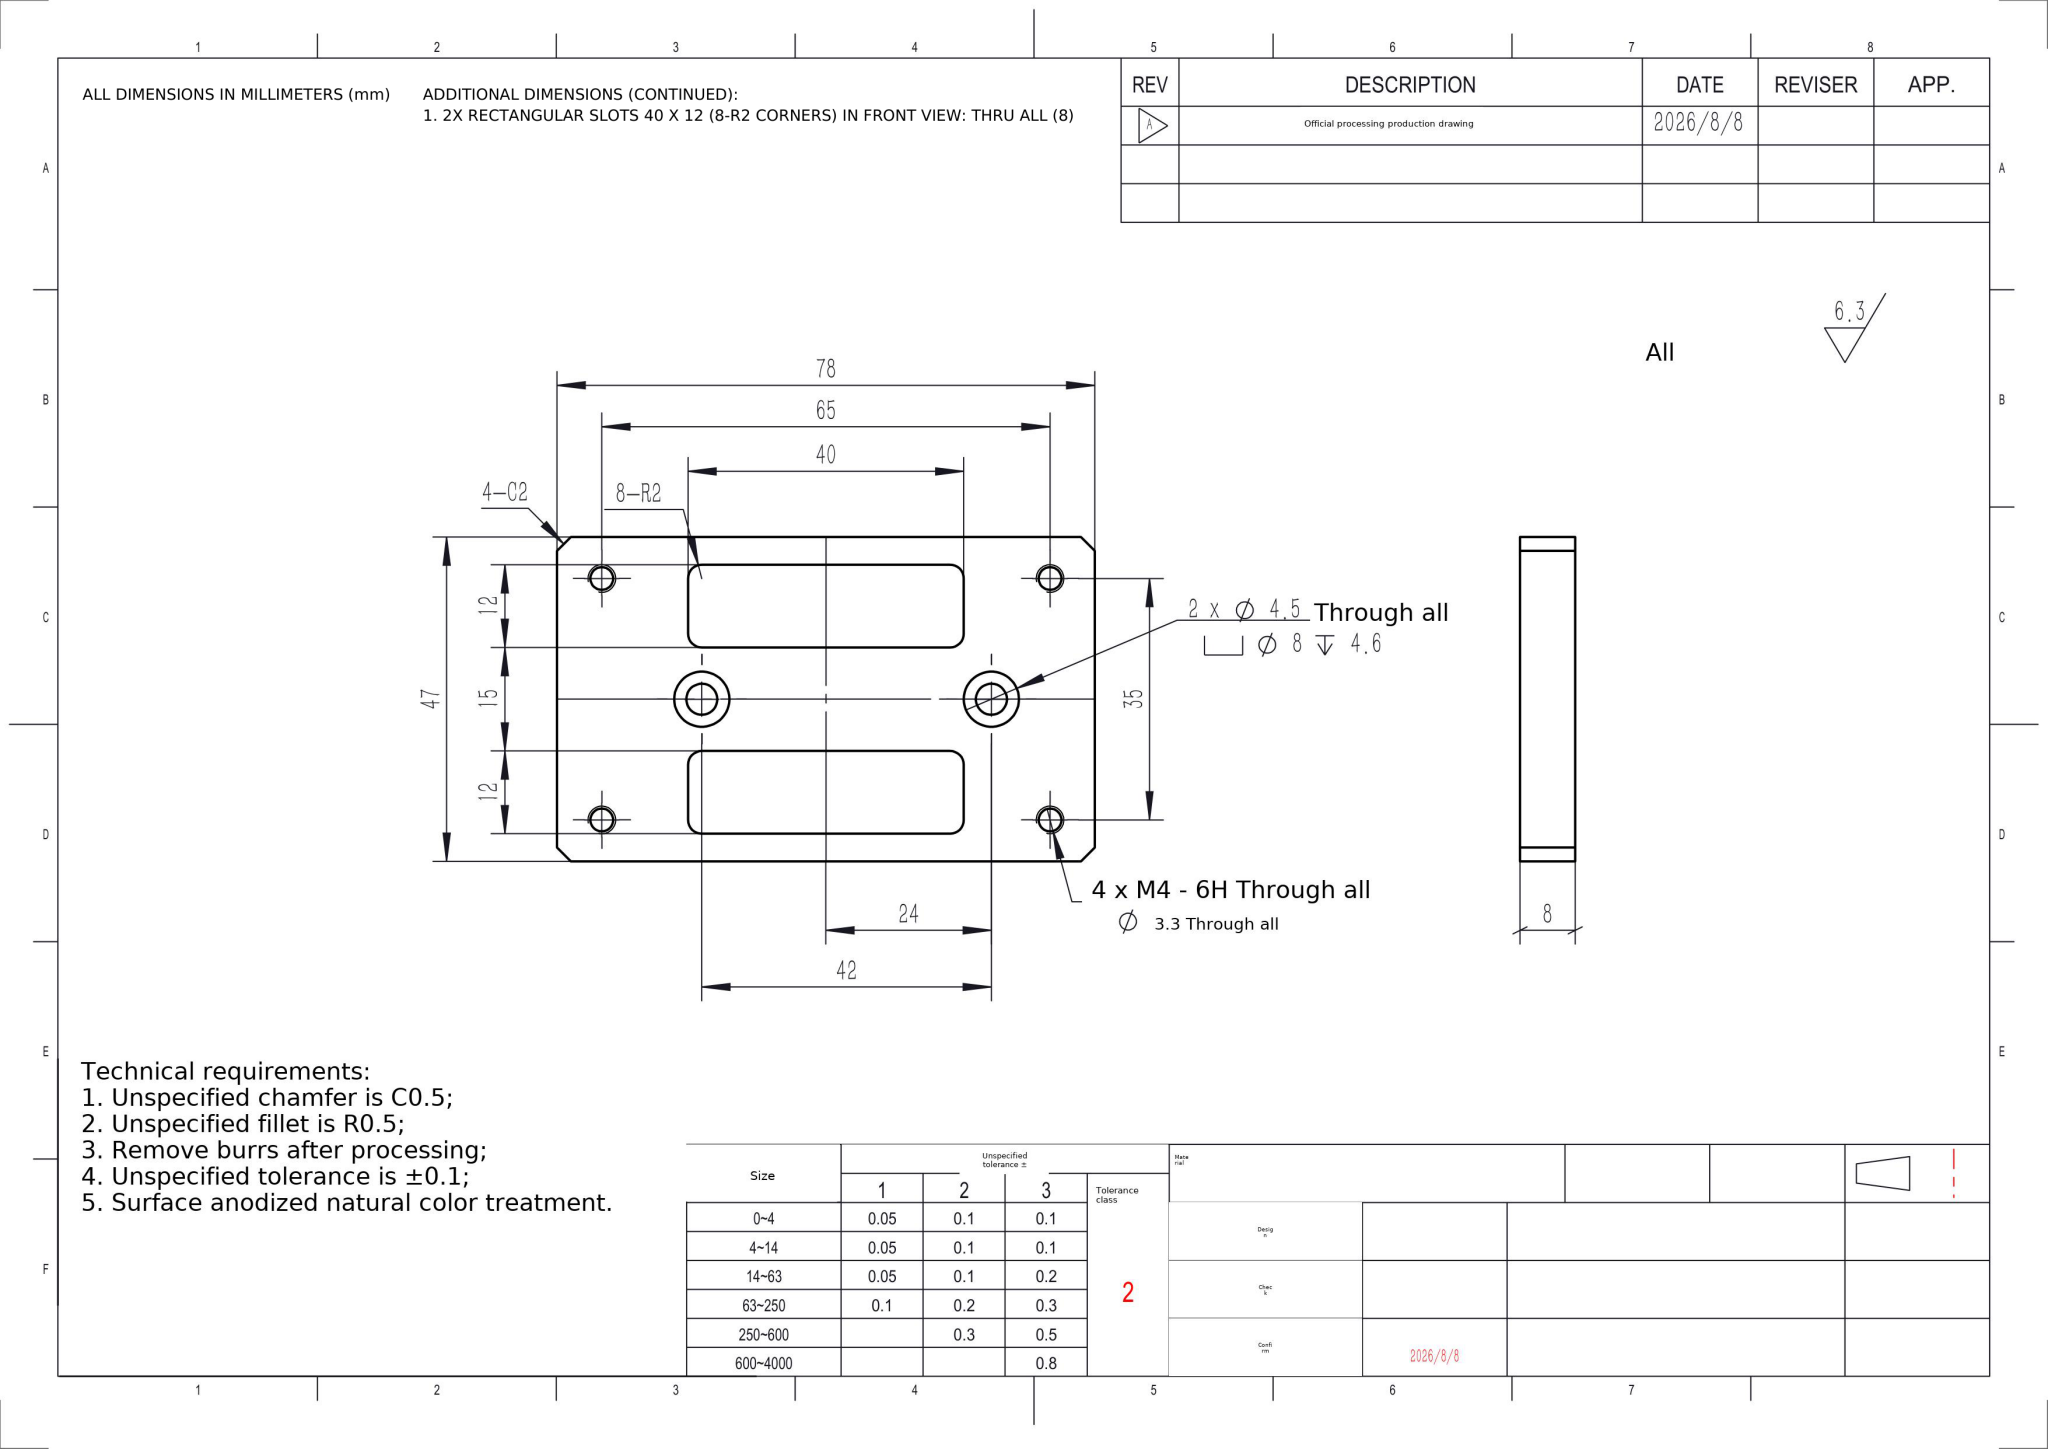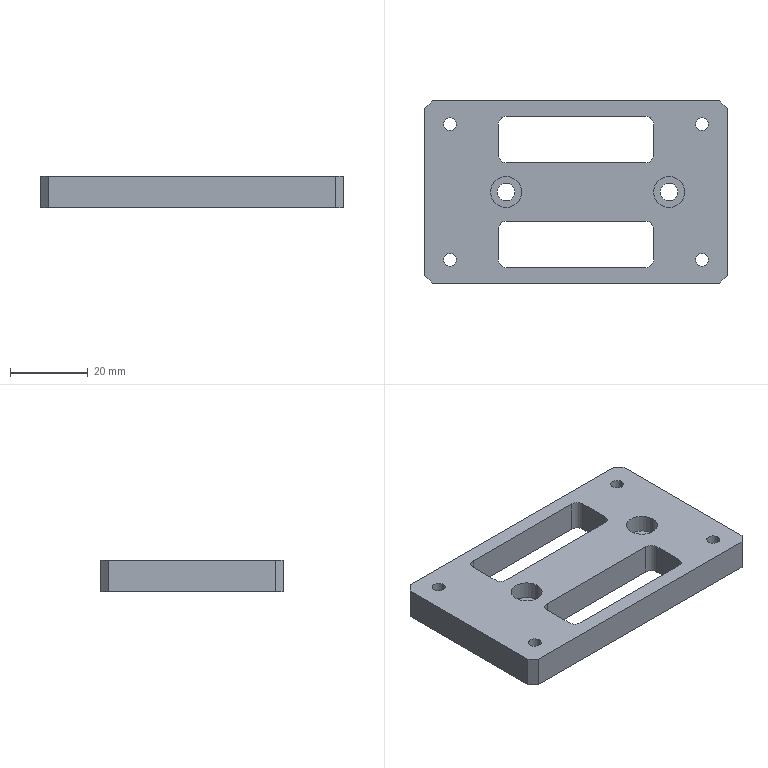Part | NX | mm | 1 solid | 44 faces | box 78 x 47 x 8 mm | volume 20795 mm3 | cylinder 24 | plane 20 | commonest cylinder face diameters 3.3 x8 4 x8 8 x4 4.5 x4